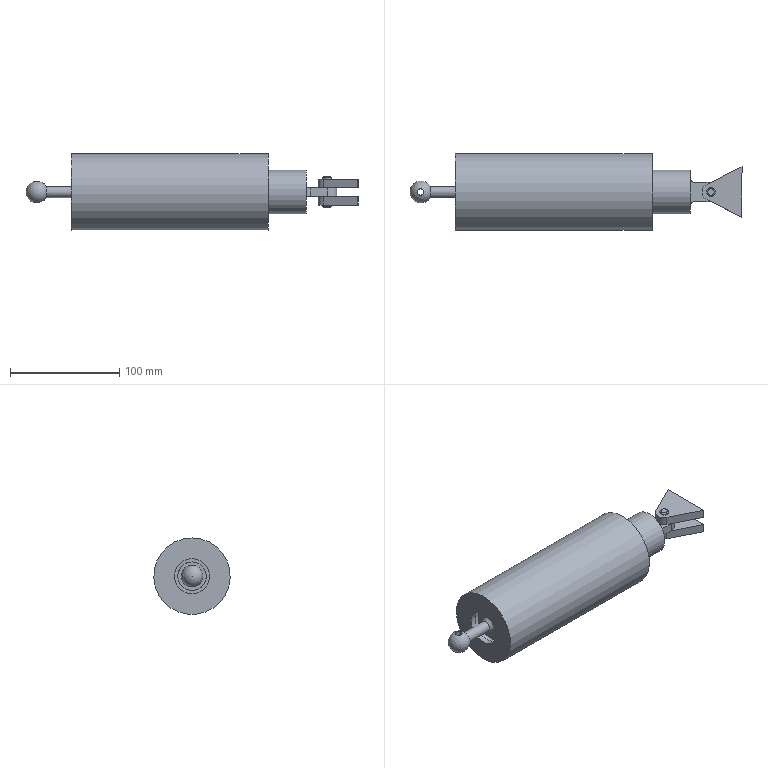Assembly | NX | mm | 11 component files | 12 solids | 85 faces | box 303.89 x 70 x 70 mm | volume 403202 mm3 | plane 46 | cylinder 32 | spline 3 | cone 3 | sphere 1 | commonest cylinder face diameters 8 x6 10 x6 26 x3 6 x2 16 x2 36 x2 52 x2 44 x2
Bill of materials:
unnamed part 1 | 1 |  | Solid cylindrical pin with a chamfer at both ends
unnamed part 2 | 2 |  | Helical coil of round-section wire with about four turns and open, unground ends
unnamed part 3 | 1 |  | Flat annular disc (washer-like ring) with a central through hole
unnamed part 4 | 1 |  | Long helical coil of thin round wire with many open-pitch turns (about 16)
unnamed part 5 | 1 |  | Stepped cylindrical body: a large cylinder, a smaller coaxial cylindrical boss, and a thin flat tab with a round end and a small hole
unnamed part 6 | 2 |  | Flat triangular plate with one rounded apex and a round through hole at that apex
unnamed part 7 | 2 |  | Flanged cylindrical bushing-like part with a thin flange at one end and a small central through bore
unnamed part 8 | 1 |  | Long slender rod with a spherical ball end containing a cross hole, and a thin collar or flange near the ball end
Mates:
1. touch align | large_spring_base 1 face | moving_rod 1 face
2. touch align | moving_rod 1 face | outer_tube 1 face
3. touch align | large_spring_base 2 face | moving_rod 1 face
4. touch align | large_spring_base 1 face | outer_tube 1 edge
5. touch align | large_spring_base 2 face | outer_tube 1 edge
6. touch align | fixed_base 2 face | outer_tube 1 face
7. touch align | pin 1 face | outer_tube 1 face